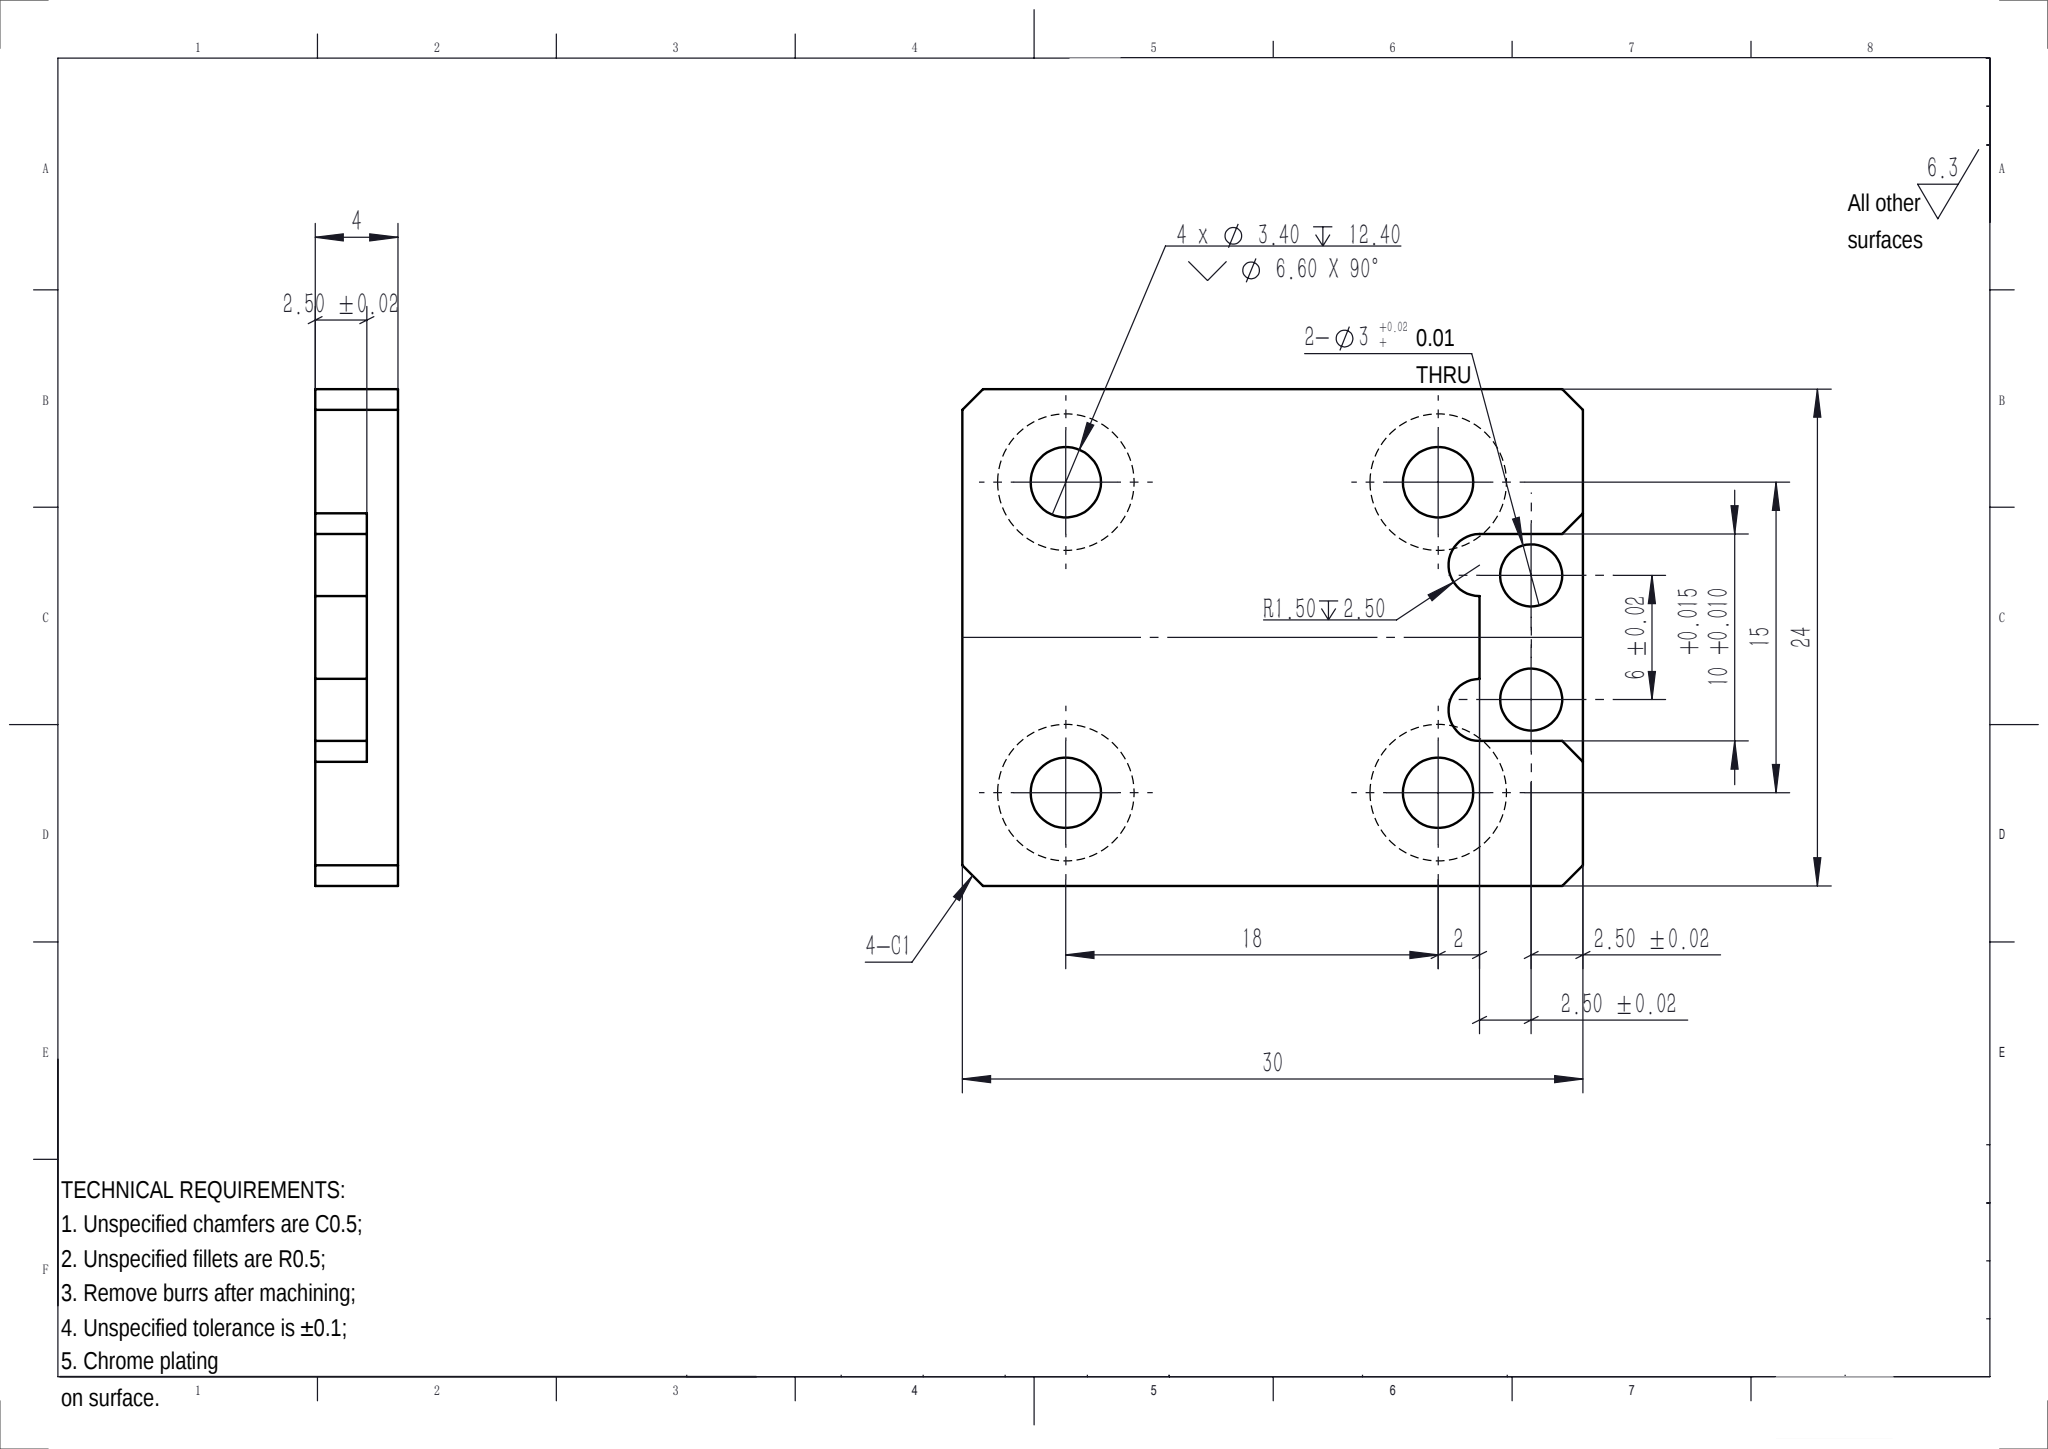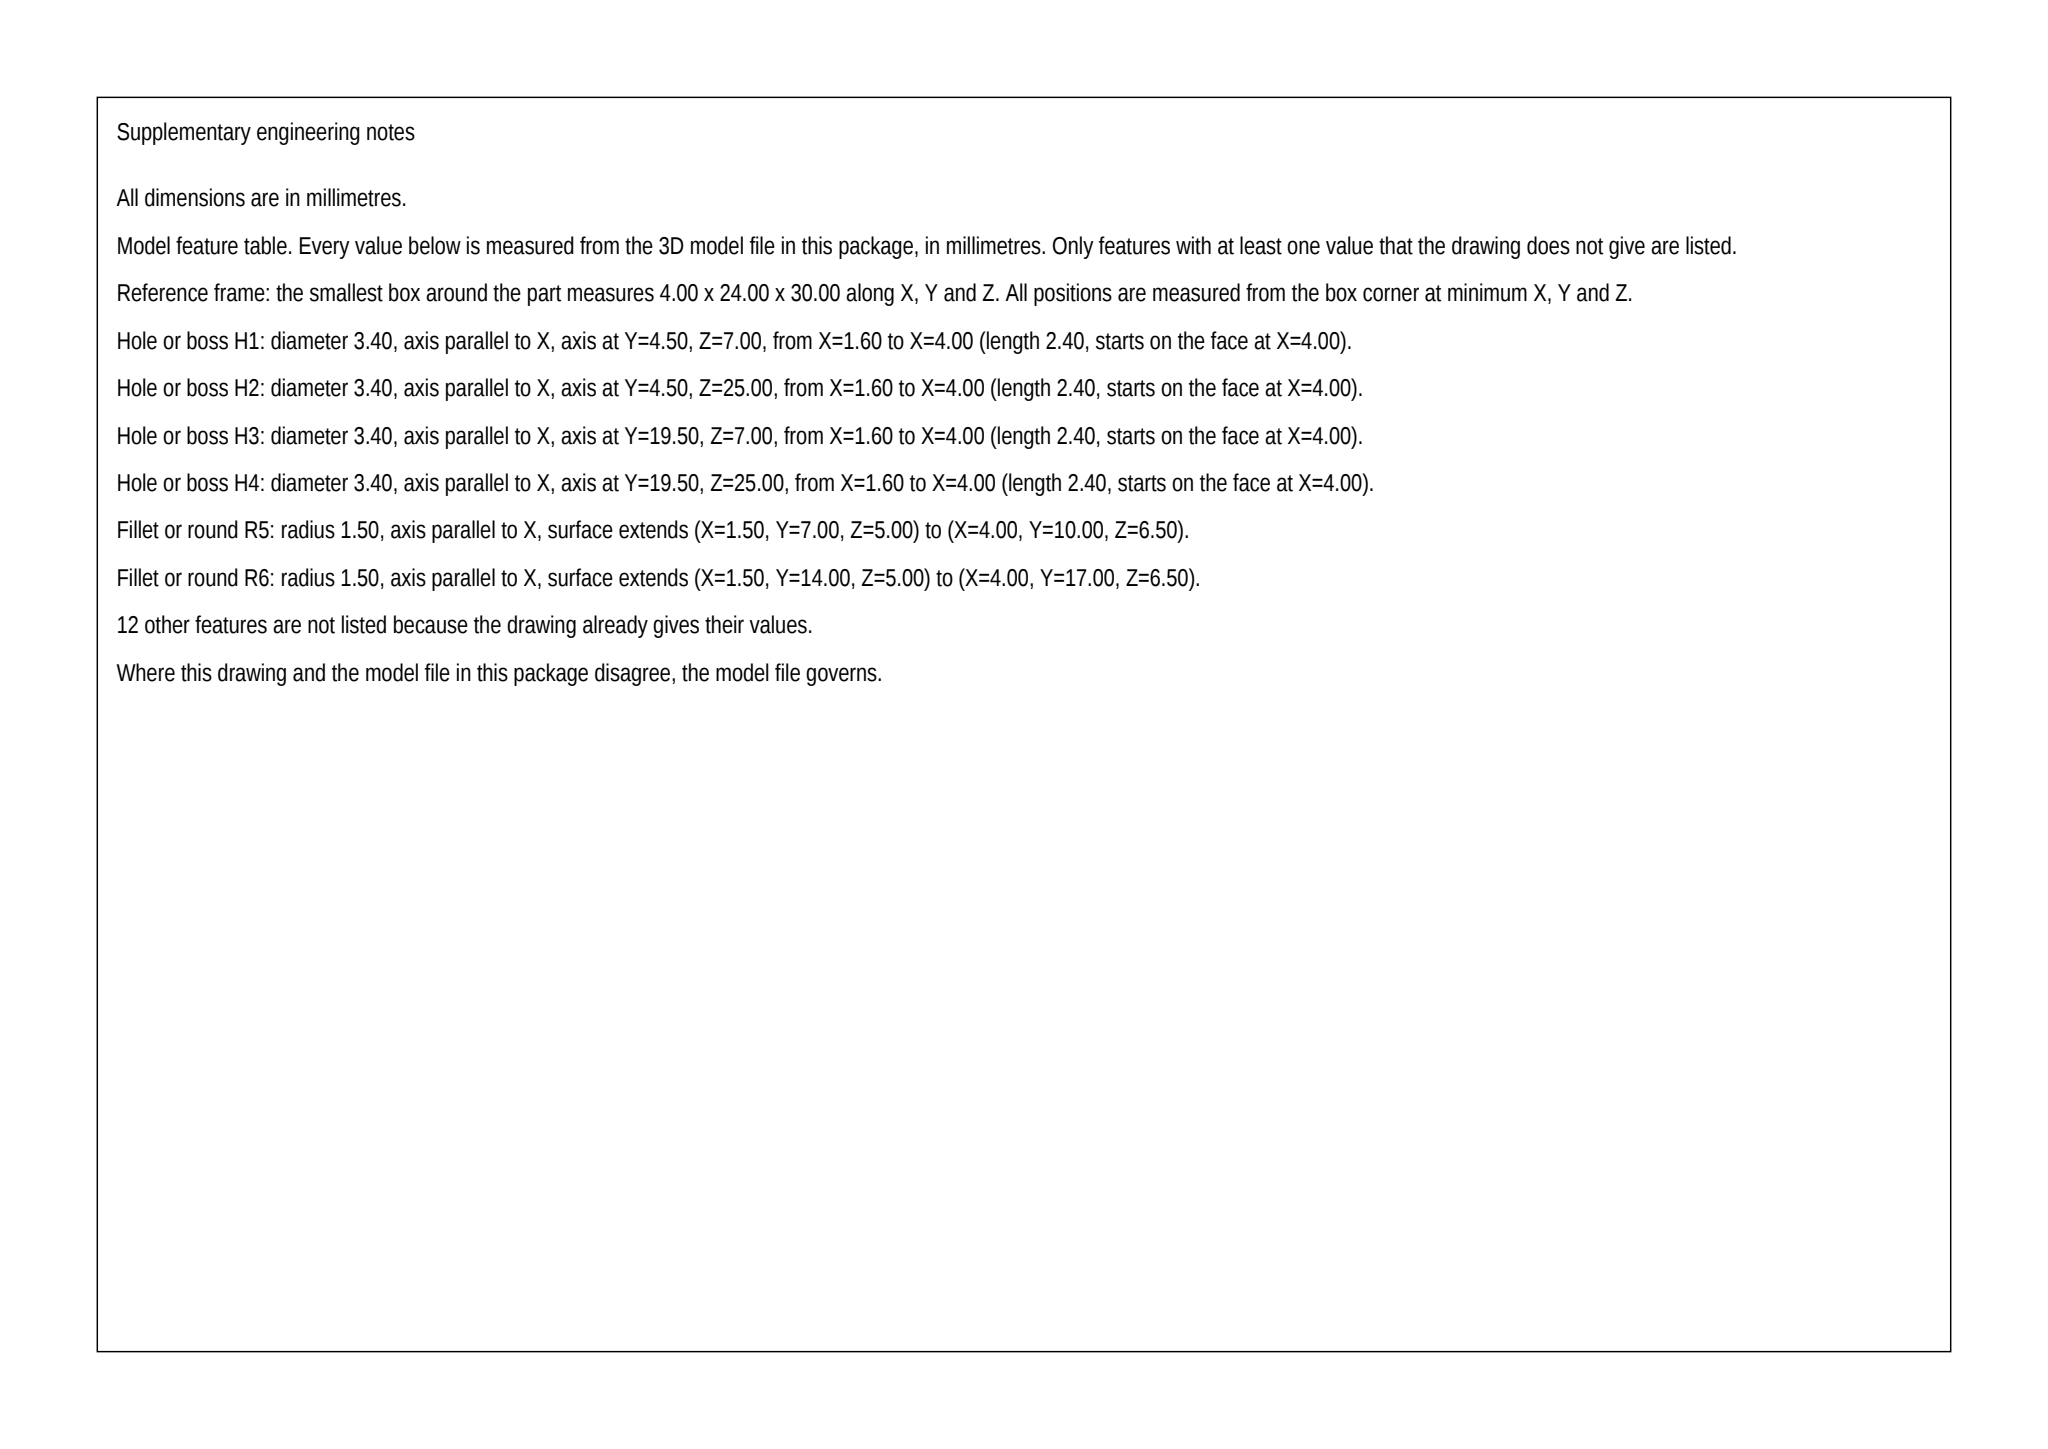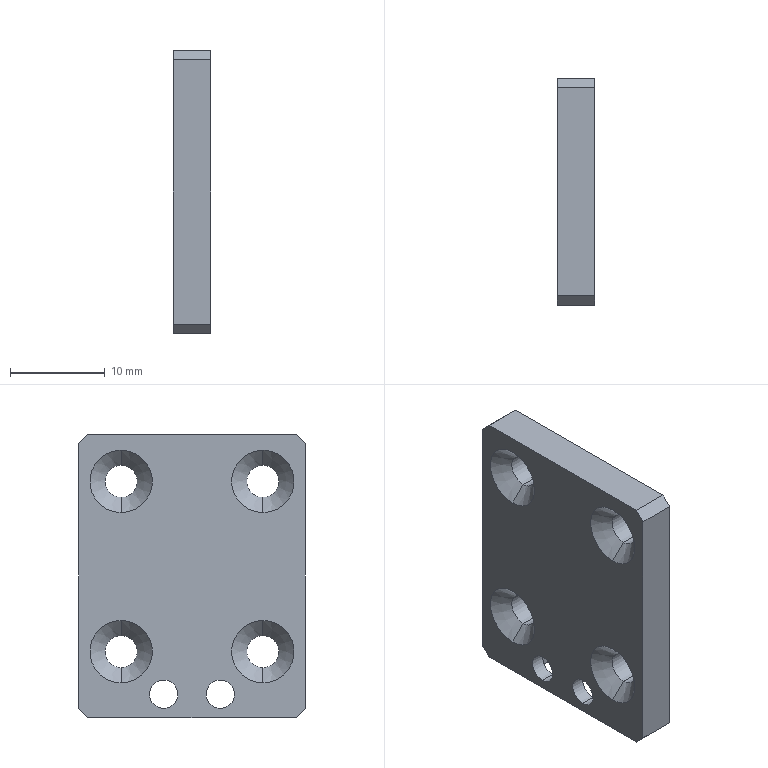Part | SolidWorks | mm | 1 solid | 38 faces | box 4 x 24 x 30 mm | volume 2489 mm3 | plane 16 | cylinder 14 | cone 8 | commonest cylinder face diameters 3.4 x8 3 x6
build123d program:
from build123d import *

# Parameters (mm, degrees)
SKETCH1_W                                         = 30
SKETCH1_H                                         = 24
BOSS_EXTRUDE1_DEPTH                               = 4
CUT_EXTRUDE1_DEPTH                                = 2.5
SKETCH3_R                                         = 1.5
CUT_EXTRUDE2_DEPTH                                = 10
HOLE_SIZE_ACCORDING_TO_PHILLIPS_RAISE_D           = 3.4
HOLE_SIZE_ACCORDING_TO_PHILLIPS_RAISE_DEPTH       = 12.4
HOLE_SIZE_ACCORDING_TO_PHILLIPS_RAISE_CSINK_D     = 6.6
HOLE_SIZE_ACCORDING_TO_PHILLIPS_RAISE_CSINK_ANGLE = 90
HOLE_SIZE_ACCORDING_TO_PHILLIPS_RAISE_TIP         = 1.021
CHAMFER1_SIZE                                     = 1


with BuildPart() as part:
    # Sketch1 → Boss-Extrude1 (new body)
    with BuildSketch(Plane(origin=(0, 0, 0), x_dir=(0, 0, -1), z_dir=(1, 0, 0))):
        Rectangle(SKETCH1_W, SKETCH1_H)
    extrude(amount=BOSS_EXTRUDE1_DEPTH)

    # Sketch2 → Cut-Extrude1 (cut)
    with BuildSketch(Plane(origin=(4, 0, 0), x_dir=(0, 0, -1), z_dir=(1, 0, 0))):
        with BuildLine():
            Line((15, 5), (10, 5))
            ThreePointArc((10, 5), (8.5, 3.5), (10, 2))
            Line((10, 2), (10, -2))
            ThreePointArc((10, -2), (8.5, -3.5), (10, -5))
            Line((10, -5), (15, -5))
            Line((15, -5), (15, 5))
        make_face()
    extrude(amount=-CUT_EXTRUDE1_DEPTH, mode=Mode.SUBTRACT)

    # Sketch3 → Cut-Extrude2 (cut)
    with BuildSketch(Plane(origin=(1.5, 0, 0), x_dir=(0, 0, -1), z_dir=(1, 0, 0))):
        with Locations((12.5, 3)):
            Circle(SKETCH3_R)
        with Locations((12.5, -3)):
            Circle(SKETCH3_R)
    extrude(amount=-CUT_EXTRUDE2_DEPTH, mode=Mode.SUBTRACT)

    # Hole Size _ according to Phillips_ Raise
    with Locations(Plane.ZY):
        with Locations((-8, 7.5), (10, 7.5), (10, -7.5), (-8, -7.5)):
            CounterSinkHole(HOLE_SIZE_ACCORDING_TO_PHILLIPS_RAISE_D / 2, HOLE_SIZE_ACCORDING_TO_PHILLIPS_RAISE_CSINK_D / 2, depth=HOLE_SIZE_ACCORDING_TO_PHILLIPS_RAISE_DEPTH, counter_sink_angle=HOLE_SIZE_ACCORDING_TO_PHILLIPS_RAISE_CSINK_ANGLE)
            with Locations((0, 0, -(HOLE_SIZE_ACCORDING_TO_PHILLIPS_RAISE_DEPTH + HOLE_SIZE_ACCORDING_TO_PHILLIPS_RAISE_TIP / 2))):  # 118° drill point
                Cone(0, HOLE_SIZE_ACCORDING_TO_PHILLIPS_RAISE_D / 2, HOLE_SIZE_ACCORDING_TO_PHILLIPS_RAISE_TIP, mode=Mode.SUBTRACT)

    # Chamfer1
    chamfer1_edges = [part.edges().sort_by_distance(p)[0] for p in [
        (2.75, 5, -15),
        (2.75, -5, -15),
        (2, -12, -15),
        (2, -12, 15),
        (2, 12, 15),
        (2, 12, -15),
    ]]
    chamfer(chamfer1_edges, length=CHAMFER1_SIZE)


solid = part.part